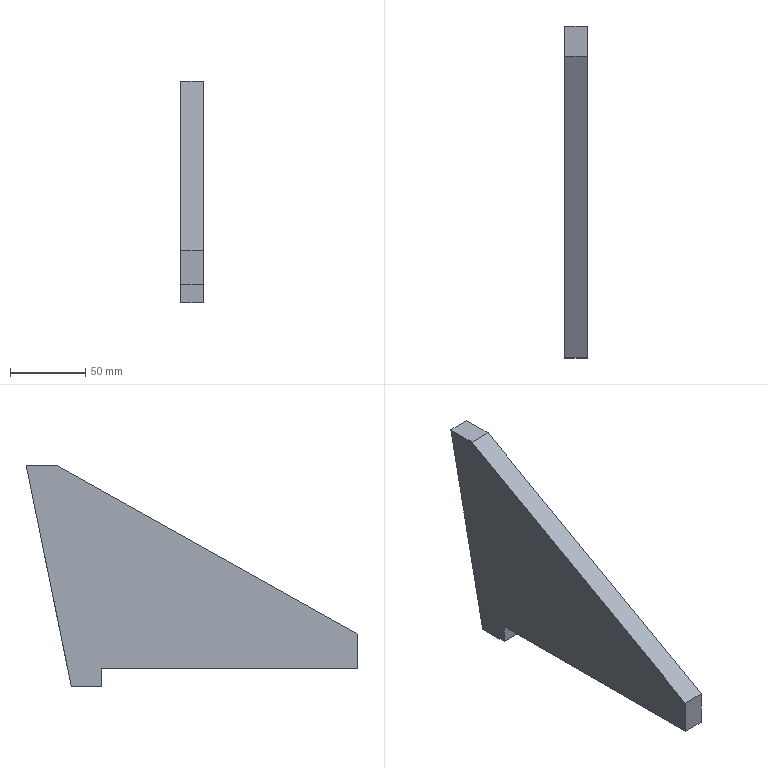Component | SolidWorks | JL001-04-01-003-1 | 1 solid | 41 faces | box 15 x 220 x 147 mm | volume 250990 mm3 | cylinder 16 | cone 16 | plane 9 | commonest cylinder face diameters 5 x16
build123d program:
from build123d import *

# Parameters (mm, degrees)
BOSS_EXTRUDE1_DEPTH   = 7.5
SKETCH2_W             = 12
SKETCH2_H             = 170
CUT_EXTRUDE1_DEPTH    = 266.017
M6_TAPPED_HOLE1_D     = 5
M6_TAPPED_HOLE1_DEPTH = 15
M6_TAPPED_HOLE1_TIP   = 1.502
M6_TAPPED_HOLE2_D     = 5
M6_TAPPED_HOLE2_DEPTH = 15
M6_TAPPED_HOLE2_TIP   = 1.502


with BuildPart() as part:
    # Sketch1 → Boss-Extrude1 (new, symmetric)
    with BuildSketch(Plane(origin=(0, 0, 0), x_dir=(0, 0, -1), z_dir=(1, 0, 0))):
        Polygon((0, 0), (0, -220), (-35, -220), (-147, -20), (-147, 0), align=None)
    extrude(amount=BOSS_EXTRUDE1_DEPTH, both=True)

    # Sketch2 → Cut-Extrude1 (cut, through all)
    with BuildSketch(Plane(origin=(7.5, 0, 0), x_dir=(0, 0, -1), z_dir=(1, 0, 0))):
        Polygon((-147, 0), (0, -30), (0, 0), align=None)
        with Locations((-6, -135)):
            Rectangle(SKETCH2_W, SKETCH2_H)
    extrude(amount=-CUT_EXTRUDE1_DEPTH, mode=Mode.SUBTRACT)

    # M6 Tapped Hole1
    with Locations(Plane(origin=(0, 0, 12), x_dir=(-1, 0, 0), z_dir=(0, 0, -1))):
        with Locations((0, -60), (0, -135), (0, -210), (0, -100), (0, -170)):
            Hole(M6_TAPPED_HOLE1_D / 2, depth=M6_TAPPED_HOLE1_DEPTH)
            with Locations((0, 0, -(M6_TAPPED_HOLE1_DEPTH + M6_TAPPED_HOLE1_TIP / 2))):  # 118° drill point
                Cone(0, M6_TAPPED_HOLE1_D / 2, M6_TAPPED_HOLE1_TIP, mode=Mode.SUBTRACT)

    # M6 Tapped Hole2
    with Locations(Plane(origin=(0, -28.8, 5.878), x_dir=(1, 0, 0), z_dir=(0, 0.9798, -0.2))):
        with Locations((0, -134.016), (0, -69.016), (0, -4.016)):
            Hole(M6_TAPPED_HOLE2_D / 2, depth=M6_TAPPED_HOLE2_DEPTH)
            with Locations((0, 0, -(M6_TAPPED_HOLE2_DEPTH + M6_TAPPED_HOLE2_TIP / 2))):  # 118° drill point
                Cone(0, M6_TAPPED_HOLE2_D / 2, M6_TAPPED_HOLE2_TIP, mode=Mode.SUBTRACT)


solid = part.part

# Placed as in the assembly
solid = solid.moved(Location((142.5, 135, 0), (0, 0, 0)))
STEP:
#1=COLOUR_RGB('',0.7922,0.8196,0.9333);
#2=FILL_AREA_STYLE_COLOUR('',#1);
#3=FILL_AREA_STYLE('',(#2));
#4=SURFACE_STYLE_FILL_AREA(#3);
#5=SURFACE_SIDE_STYLE('',(#4));
#6=SURFACE_STYLE_USAGE(.BOTH.,#5);
#7=PRESENTATION_STYLE_ASSIGNMENT((#6));
#8=CARTESIAN_POINT('',(5.61,4.638,5.423));
#9=VERTEX_POINT('',#8);
#10=CARTESIAN_POINT('',(5.61,4.677,5.616));
#11=VERTEX_POINT('',#10);
#12=CARTESIAN_POINT('',(5.61,4.657,5.519));
#13=DIRECTION('',(0.,0.9798,-0.2));
#14=DIRECTION('',(0.,0.2,0.9798));
#15=AXIS2_PLACEMENT_3D('',#12,#13,#14);
#16=CIRCLE('',#15,0.09843);
#17=EDGE_CURVE('',#9,#11,#16,.T.);
#18=ORIENTED_EDGE('',*,*,#17,.F.);
#19=CARTESIAN_POINT('',(5.61,5.216,5.305));
#20=VERTEX_POINT('',#19);
#21=CARTESIAN_POINT('',(5.61,5.216,5.305));
#22=DIRECTION('',(0.,0.9798,-0.2));
#23=VECTOR('',#22,39.37);
#24=LINE('',#21,#23);
#25=EDGE_CURVE('',#9,#20,#24,.T.);
#26=ORIENTED_EDGE('',*,*,#25,.T.);
#27=CARTESIAN_POINT('',(5.61,5.256,5.498));
#28=VERTEX_POINT('',#27);
#29=CARTESIAN_POINT('',(5.61,5.236,5.401));
#30=DIRECTION('',(0.,0.9798,-0.2));
#31=DIRECTION('',(0.,0.2,0.9798));
#32=AXIS2_PLACEMENT_3D('',#29,#30,#31);
#33=CIRCLE('',#32,0.09843);
#34=EDGE_CURVE('',#20,#28,#33,.T.);
#35=ORIENTED_EDGE('',*,*,#34,.T.);
#36=CARTESIAN_POINT('',(5.61,5.256,5.498));
#37=DIRECTION('',(0.,0.9798,-0.2));
#38=VECTOR('',#37,39.37);
#39=LINE('',#36,#38);
#40=EDGE_CURVE('',#11,#28,#39,.T.);
#41=ORIENTED_EDGE('',*,*,#40,.F.);
#42=EDGE_LOOP('',(#18,#26,#35,#41));
#43=FACE_OUTER_BOUND('',#42,.T.);
#44=CARTESIAN_POINT('',(5.61,5.236,5.401));
#45=DIRECTION('',(0.,0.9798,-0.2));
#46=DIRECTION('',(0.,0.2,0.9798));
#47=AXIS2_PLACEMENT_3D('',#44,#45,#46);
#48=CYLINDRICAL_SURFACE('',#47,0.09843);
#49=ADVANCED_FACE('',(#43),#48,.F.);
#50=CARTESIAN_POINT('',(5.61,4.6,5.531));
#51=VERTEX_POINT('',#50);
#52=CARTESIAN_POINT('',(5.61,4.677,5.616));
#53=DIRECTION('',(0.,0.676,0.7369));
#54=VECTOR('',#53,39.37);
#55=LINE('',#52,#54);
#56=EDGE_CURVE('',#51,#11,#55,.T.);
#57=ORIENTED_EDGE('',*,*,#56,.F.);
#58=CARTESIAN_POINT('',(5.61,4.638,5.423));
#59=DIRECTION('',(0.,0.3332,-0.9428));
#60=VECTOR('',#59,39.37);
#61=LINE('',#58,#60);
#62=EDGE_CURVE('',#51,#9,#61,.T.);
#63=ORIENTED_EDGE('',*,*,#62,.T.);
#64=ORIENTED_EDGE('',*,*,#17,.T.);
#65=EDGE_LOOP('',(#57,#63,#64));
#66=FACE_OUTER_BOUND('',#65,.T.);
#67=CARTESIAN_POINT('',(5.61,4.657,5.519));
#68=DIRECTION('',(0.,0.9798,-0.2));
#69=DIRECTION('',(0.,0.2,0.9798));
#70=AXIS2_PLACEMENT_3D('',#67,#68,#69);
#71=CONICAL_SURFACE('',#70,0.09843,1.03);
#72=ADVANCED_FACE('',(#66),#71,.F.);
#73=CARTESIAN_POINT('',(5.61,4.126,2.915));
#74=VERTEX_POINT('',#73);
#75=CARTESIAN_POINT('',(5.61,4.165,3.108));
#76=VERTEX_POINT('',#75);
#77=CARTESIAN_POINT('',(5.61,4.146,3.012));
#78=DIRECTION('',(0.,0.9798,-0.2));
#79=DIRECTION('',(0.,0.2,0.9798));
#80=AXIS2_PLACEMENT_3D('',#77,#78,#79);
#81=CIRCLE('',#80,0.09843);
#82=EDGE_CURVE('',#74,#76,#81,.T.);
#83=ORIENTED_EDGE('',*,*,#82,.F.);
#84=CARTESIAN_POINT('',(5.61,4.705,2.797));
#85=VERTEX_POINT('',#84);
#86=CARTESIAN_POINT('',(5.61,4.705,2.797));
#87=DIRECTION('',(0.,0.9798,-0.2));
#88=VECTOR('',#87,39.37);
#89=LINE('',#86,#88);
#90=EDGE_CURVE('',#74,#85,#89,.T.);
#91=ORIENTED_EDGE('',*,*,#90,.T.);
#92=CARTESIAN_POINT('',(5.61,4.744,2.99));
#93=VERTEX_POINT('',#92);
#94=CARTESIAN_POINT('',(5.61,4.724,2.894));
#95=DIRECTION('',(0.,0.9798,-0.2));
#96=DIRECTION('',(0.,0.2,0.9798));
#97=AXIS2_PLACEMENT_3D('',#94,#95,#96);
#98=CIRCLE('',#97,0.09843);
#99=EDGE_CURVE('',#85,#93,#98,.T.);
#100=ORIENTED_EDGE('',*,*,#99,.T.);
#101=CARTESIAN_POINT('',(5.61,4.744,2.99));
#102=DIRECTION('',(0.,0.9798,-0.2));
#103=VECTOR('',#102,39.37);
#104=LINE('',#101,#103);
#105=EDGE_CURVE('',#76,#93,#104,.T.);
#106=ORIENTED_EDGE('',*,*,#105,.F.);
#107=EDGE_LOOP('',(#83,#91,#100,#106));
#108=FACE_OUTER_BOUND('',#107,.T.);
#109=CARTESIAN_POINT('',(5.61,4.724,2.894));
#110=DIRECTION('',(0.,0.9798,-0.2));
#111=DIRECTION('',(0.,0.2,0.9798));
#112=AXIS2_PLACEMENT_3D('',#109,#110,#111);
#113=CYLINDRICAL_SURFACE('',#112,0.09843);
#114=ADVANCED_FACE('',(#108),#113,.F.);
#115=CARTESIAN_POINT('',(5.61,4.088,3.024));
#116=VERTEX_POINT('',#115);
#117=CARTESIAN_POINT('',(5.61,4.165,3.108));
#118=DIRECTION('',(0.,0.676,0.7369));
#119=VECTOR('',#118,39.37);
#120=LINE('',#117,#119);
#121=EDGE_CURVE('',#116,#76,#120,.T.);
#122=ORIENTED_EDGE('',*,*,#121,.F.);
#123=CARTESIAN_POINT('',(5.61,4.126,2.915));
#124=DIRECTION('',(0.,0.3332,-0.9428));
#125=VECTOR('',#124,39.37);
#126=LINE('',#123,#125);
#127=EDGE_CURVE('',#116,#74,#126,.T.);
#128=ORIENTED_EDGE('',*,*,#127,.T.);
#129=ORIENTED_EDGE('',*,*,#82,.T.);
#130=EDGE_LOOP('',(#122,#128,#129));
#131=FACE_OUTER_BOUND('',#130,.T.);
#132=CARTESIAN_POINT('',(5.61,4.146,3.012));
#133=DIRECTION('',(0.,0.9798,-0.2));
#134=DIRECTION('',(0.,0.2,0.9798));
#135=AXIS2_PLACEMENT_3D('',#132,#133,#134);
#136=CONICAL_SURFACE('',#135,0.09843,1.03);
#137=ADVANCED_FACE('',(#131),#136,.F.);
#138=CARTESIAN_POINT('',(5.61,3.614,0.408));
#139=VERTEX_POINT('',#138);
#140=CARTESIAN_POINT('',(5.61,3.654,0.6009));
#141=VERTEX_POINT('',#140);
#142=CARTESIAN_POINT('',(5.61,3.634,0.5044));
#143=DIRECTION('',(0.,0.9798,-0.2));
#144=DIRECTION('',(0.,0.2,0.9798));
#145=AXIS2_PLACEMENT_3D('',#142,#143,#144);
#146=CIRCLE('',#145,0.09843);
#147=EDGE_CURVE('',#139,#141,#146,.T.);
#148=ORIENTED_EDGE('',*,*,#147,.F.);
#149=CARTESIAN_POINT('',(5.61,4.193,0.2899));
#150=VERTEX_POINT('',#149);
#151=CARTESIAN_POINT('',(5.61,4.193,0.2899));
#152=DIRECTION('',(0.,0.9798,-0.2));
#153=VECTOR('',#152,39.37);
#154=LINE('',#151,#153);
#155=EDGE_CURVE('',#139,#150,#154,.T.);
#156=ORIENTED_EDGE('',*,*,#155,.T.);
#157=CARTESIAN_POINT('',(5.61,4.232,0.4828));
#158=VERTEX_POINT('',#157);
#159=CARTESIAN_POINT('',(5.61,4.213,0.3863));
#160=DIRECTION('',(0.,0.9798,-0.2));
#161=DIRECTION('',(0.,0.2,0.9798));
#162=AXIS2_PLACEMENT_3D('',#159,#160,#161);
#163=CIRCLE('',#162,0.09843);
#164=EDGE_CURVE('',#150,#158,#163,.T.);
#165=ORIENTED_EDGE('',*,*,#164,.T.);
#166=CARTESIAN_POINT('',(5.61,4.232,0.4828));
#167=DIRECTION('',(0.,0.9798,-0.2));
#168=VECTOR('',#167,39.37);
#169=LINE('',#166,#168);
#170=EDGE_CURVE('',#141,#158,#169,.T.);
#171=ORIENTED_EDGE('',*,*,#170,.F.);
#172=EDGE_LOOP('',(#148,#156,#165,#171));
#173=FACE_OUTER_BOUND('',#172,.T.);
#174=CARTESIAN_POINT('',(5.61,4.213,0.3863));
#175=DIRECTION('',(0.,0.9798,-0.2));
#176=DIRECTION('',(0.,0.2,0.9798));
#177=AXIS2_PLACEMENT_3D('',#174,#175,#176);
#178=CYLINDRICAL_SURFACE('',#177,0.09843);
#179=ADVANCED_FACE('',(#173),#178,.F.);
#180=CARTESIAN_POINT('',(5.61,3.576,0.5162));
#181=VERTEX_POINT('',#180);
#182=CARTESIAN_POINT('',(5.61,3.654,0.6009));
#183=DIRECTION('',(0.,0.676,0.7369));
#184=VECTOR('',#183,39.37);
#185=LINE('',#182,#184);
#186=EDGE_CURVE('',#181,#141,#185,.T.);
#187=ORIENTED_EDGE('',*,*,#186,.F.);
#188=CARTESIAN_POINT('',(5.61,3.614,0.408));
#189=DIRECTION('',(0.,0.3332,-0.9428));
#190=VECTOR('',#189,39.37);
#191=LINE('',#188,#190);
#192=EDGE_CURVE('',#181,#139,#191,.T.);
#193=ORIENTED_EDGE('',*,*,#192,.T.);
#194=ORIENTED_EDGE('',*,*,#147,.T.);
#195=EDGE_LOOP('',(#187,#193,#194));
#196=FACE_OUTER_BOUND('',#195,.T.);
#197=CARTESIAN_POINT('',(5.61,3.634,0.5044));
#198=DIRECTION('',(0.,0.9798,-0.2));
#199=DIRECTION('',(0.,0.2,0.9798));
#200=AXIS2_PLACEMENT_3D('',#197,#198,#199);
#201=CONICAL_SURFACE('',#200,0.09843,1.03);
#202=ADVANCED_FACE('',(#196),#201,.F.);
#203=CARTESIAN_POINT('',(5.61,2.854,1.063));
#204=VERTEX_POINT('',#203);
#205=CARTESIAN_POINT('',(5.61,3.051,1.063));
#206=VERTEX_POINT('',#205);
#207=CARTESIAN_POINT('',(5.61,2.953,1.063));
#208=DIRECTION('',(0.,0.,-1.));
#209=DIRECTION('',(0.,1.,0.));
#210=AXIS2_PLACEMENT_3D('',#207,#208,#209);
#211=CIRCLE('',#210,0.09843);
#212=EDGE_CURVE('',#204,#206,#211,.T.);
#213=ORIENTED_EDGE('',*,*,#212,.F.);
#214=CARTESIAN_POINT('',(5.61,2.854,0.4724));
#215=VERTEX_POINT('',#214);
#216=CARTESIAN_POINT('',(5.61,2.854,0.4724));
#217=DIRECTION('',(0.,0.,-1.));
#218=VECTOR('',#217,39.37);
#219=LINE('',#216,#218);
#220=EDGE_CURVE('',#204,#215,#219,.T.);
#221=ORIENTED_EDGE('',*,*,#220,.T.);
#222=CARTESIAN_POINT('',(5.61,3.051,0.4724));
#223=VERTEX_POINT('',#222);
#224=CARTESIAN_POINT('',(5.61,2.953,0.4724));
#225=DIRECTION('',(0.,0.,-1.));
#226=DIRECTION('',(0.,1.,0.));
#227=AXIS2_PLACEMENT_3D('',#224,#225,#226);
#228=CIRCLE('',#227,0.09843);
#229=EDGE_CURVE('',#215,#223,#228,.T.);
#230=ORIENTED_EDGE('',*,*,#229,.T.);
#231=CARTESIAN_POINT('',(5.61,3.051,0.4724));
#232=DIRECTION('',(0.,0.,-1.));
#233=VECTOR('',#232,39.37);
#234=LINE('',#231,#233);
#235=EDGE_CURVE('',#206,#223,#234,.T.);
#236=ORIENTED_EDGE('',*,*,#235,.F.);
#237=EDGE_LOOP('',(#213,#221,#230,#236));
#238=FACE_OUTER_BOUND('',#237,.T.);
#239=CARTESIAN_POINT('',(5.61,2.953,0.4724));
#240=DIRECTION('',(0.,0.,-1.));
#241=DIRECTION('',(0.,1.,0.));
#242=AXIS2_PLACEMENT_3D('',#239,#240,#241);
#243=CYLINDRICAL_SURFACE('',#242,0.09843);
#244=ADVANCED_FACE('',(#238),#243,.F.);
#245=CARTESIAN_POINT('',(5.61,2.953,1.122));
#246=VERTEX_POINT('',#245);
#247=CARTESIAN_POINT('',(5.61,3.051,1.063));
#248=DIRECTION('',(0.,0.8572,-0.515));
#249=VECTOR('',#248,39.37);
#250=LINE('',#247,#249);
#251=EDGE_CURVE('',#246,#206,#250,.T.);
#252=ORIENTED_EDGE('',*,*,#251,.F.);
#253=CARTESIAN_POINT('',(5.61,2.854,1.063));
#254=DIRECTION('',(0.,-0.8572,-0.515));
#255=VECTOR('',#254,39.37);
#256=LINE('',#253,#255);
#257=EDGE_CURVE('',#246,#204,#256,.T.);
#258=ORIENTED_EDGE('',*,*,#257,.T.);
#259=ORIENTED_EDGE('',*,*,#212,.T.);
#260=EDGE_LOOP('',(#252,#258,#259));
#261=FACE_OUTER_BOUND('',#260,.T.);
#262=CARTESIAN_POINT('',(5.61,2.953,1.063));
#263=DIRECTION('',(0.,0.,-1.));
#264=DIRECTION('',(0.,1.,0.));
#265=AXIS2_PLACEMENT_3D('',#262,#263,#264);
#266=CONICAL_SURFACE('',#265,0.09843,1.03);
#267=ADVANCED_FACE('',(#261),#266,.F.);
#268=CARTESIAN_POINT('',(5.61,-0.09843,1.063));
#269=VERTEX_POINT('',#268);
#270=CARTESIAN_POINT('',(5.61,0.09843,1.063));
#271=VERTEX_POINT('',#270);
#272=CARTESIAN_POINT('',(5.61,0.,1.063));
#273=DIRECTION('',(0.,0.,-1.));
#274=DIRECTION('',(0.,1.,0.));
#275=AXIS2_PLACEMENT_3D('',#272,#273,#274);
#276=CIRCLE('',#275,0.09843);
#277=EDGE_CURVE('',#269,#271,#276,.T.);
#278=ORIENTED_EDGE('',*,*,#277,.F.);
#279=CARTESIAN_POINT('',(5.61,-0.09843,0.4724));
#280=VERTEX_POINT('',#279);
#281=CARTESIAN_POINT('',(5.61,-0.09843,0.4724));
#282=DIRECTION('',(0.,0.,-1.));
#283=VECTOR('',#282,39.37);
#284=LINE('',#281,#283);
#285=EDGE_CURVE('',#269,#280,#284,.T.);
#286=ORIENTED_EDGE('',*,*,#285,.T.);
#287=CARTESIAN_POINT('',(5.61,0.09843,0.4724));
#288=VERTEX_POINT('',#287);
#289=CARTESIAN_POINT('',(5.61,0.,0.4724));
#290=DIRECTION('',(0.,0.,-1.));
#291=DIRECTION('',(0.,1.,0.));
#292=AXIS2_PLACEMENT_3D('',#289,#290,#291);
#293=CIRCLE('',#292,0.09843);
#294=EDGE_CURVE('',#280,#288,#293,.T.);
#295=ORIENTED_EDGE('',*,*,#294,.T.);
#296=CARTESIAN_POINT('',(5.61,0.09843,0.4724));
#297=DIRECTION('',(0.,0.,-1.));
#298=VECTOR('',#297,39.37);
#299=LINE('',#296,#298);
#300=EDGE_CURVE('',#271,#288,#299,.T.);
#301=ORIENTED_EDGE('',*,*,#300,.F.);
#302=EDGE_LOOP('',(#278,#286,#295,#301));
#303=FACE_OUTER_BOUND('',#302,.T.);
#304=CARTESIAN_POINT('',(5.61,0.,0.4724));
#305=DIRECTION('',(0.,0.,-1.));
#306=DIRECTION('',(0.,1.,0.));
#307=AXIS2_PLACEMENT_3D('',#304,#305,#306);
#308=CYLINDRICAL_SURFACE('',#307,0.09843);
#309=ADVANCED_FACE('',(#303),#308,.F.);
#310=CARTESIAN_POINT('',(5.61,0.,1.122));
#311=VERTEX_POINT('',#310);
#312=CARTESIAN_POINT('',(5.61,0.09843,1.063));
#313=DIRECTION('',(0.,0.8572,-0.515));
#314=VECTOR('',#313,39.37);
#315=LINE('',#312,#314);
#316=EDGE_CURVE('',#311,#271,#315,.T.);
#317=ORIENTED_EDGE('',*,*,#316,.F.);
#318=CARTESIAN_POINT('',(5.61,-0.09843,1.063));
#319=DIRECTION('',(0.,-0.8572,-0.515));
#320=VECTOR('',#319,39.37);
#321=LINE('',#318,#320);
#322=EDGE_CURVE('',#311,#269,#321,.T.);
#323=ORIENTED_EDGE('',*,*,#322,.T.);
#324=ORIENTED_EDGE('',*,*,#277,.T.);
#325=EDGE_LOOP('',(#317,#323,#324));
#326=FACE_OUTER_BOUND('',#325,.T.);
#327=CARTESIAN_POINT('',(5.61,0.,1.063));
#328=DIRECTION('',(0.,0.,-1.));
#329=DIRECTION('',(0.,1.,0.));
#330=AXIS2_PLACEMENT_3D('',#327,#328,#329);
#331=CONICAL_SURFACE('',#330,0.09843,1.03);
#332=ADVANCED_FACE('',(#326),#331,.F.);
#333=CARTESIAN_POINT('',(5.61,-3.051,1.063));
#334=VERTEX_POINT('',#333);
#335=CARTESIAN_POINT('',(5.61,-2.854,1.063));
#336=VERTEX_POINT('',#335);
#337=CARTESIAN_POINT('',(5.61,-2.953,1.063));
#338=DIRECTION('',(0.,0.,-1.));
#339=DIRECTION('',(0.,1.,0.));
#340=AXIS2_PLACEMENT_3D('',#337,#338,#339);
#341=CIRCLE('',#340,0.09843);
#342=EDGE_CURVE('',#334,#336,#341,.T.);
#343=ORIENTED_EDGE('',*,*,#342,.F.);
#344=CARTESIAN_POINT('',(5.61,-3.051,0.4724));
#345=VERTEX_POINT('',#344);
#346=CARTESIAN_POINT('',(5.61,-3.051,0.4724));
#347=DIRECTION('',(0.,0.,-1.));
#348=VECTOR('',#347,39.37);
#349=LINE('',#346,#348);
#350=EDGE_CURVE('',#334,#345,#349,.T.);
#351=ORIENTED_EDGE('',*,*,#350,.T.);
#352=CARTESIAN_POINT('',(5.61,-2.854,0.4724));
#353=VERTEX_POINT('',#352);
#354=CARTESIAN_POINT('',(5.61,-2.953,0.4724));
#355=DIRECTION('',(0.,0.,-1.));
#356=DIRECTION('',(0.,1.,0.));
#357=AXIS2_PLACEMENT_3D('',#354,#355,#356);
#358=CIRCLE('',#357,0.09843);
#359=EDGE_CURVE('',#345,#353,#358,.T.);
#360=ORIENTED_EDGE('',*,*,#359,.T.);
#361=CARTESIAN_POINT('',(5.61,-2.854,0.4724));
#362=DIRECTION('',(0.,0.,-1.));
#363=VECTOR('',#362,39.37);
#364=LINE('',#361,#363);
#365=EDGE_CURVE('',#336,#353,#364,.T.);
#366=ORIENTED_EDGE('',*,*,#365,.F.);
#367=EDGE_LOOP('',(#343,#351,#360,#366));
#368=FACE_OUTER_BOUND('',#367,.T.);
#369=CARTESIAN_POINT('',(5.61,-2.953,0.4724));
#370=DIRECTION('',(0.,0.,-1.));
#371=DIRECTION('',(0.,1.,0.));
#372=AXIS2_PLACEMENT_3D('',#369,#370,#371);
#373=CYLINDRICAL_SURFACE('',#372,0.09843);
#374=ADVANCED_FACE('',(#368),#373,.F.);
#375=CARTESIAN_POINT('',(5.61,-2.953,1.122));
#376=VERTEX_POINT('',#375);
#377=CARTESIAN_POINT('',(5.61,-2.854,1.063));
#378=DIRECTION('',(0.,0.8572,-0.515));
#379=VECTOR('',#378,39.37);
#380=LINE('',#377,#379);
#381=EDGE_CURVE('',#376,#336,#380,.T.);
#382=ORIENTED_EDGE('',*,*,#381,.F.);
#383=CARTESIAN_POINT('',(5.61,-3.051,1.063));
#384=DIRECTION('',(0.,-0.8572,-0.515));
#385=VECTOR('',#384,39.37);
#386=LINE('',#383,#385);
#387=EDGE_CURVE('',#376,#334,#386,.T.);
#388=ORIENTED_EDGE('',*,*,#387,.T.);
#389=ORIENTED_EDGE('',*,*,#342,.T.);
#390=EDGE_LOOP('',(#382,#388,#389));
#391=FACE_OUTER_BOUND('',#390,.T.);
#392=CARTESIAN_POINT('',(5.61,-2.953,1.063));
#393=DIRECTION('',(0.,0.,-1.));
#394=DIRECTION('',(0.,1.,0.));
#395=AXIS2_PLACEMENT_3D('',#392,#393,#394);
#396=CONICAL_SURFACE('',#395,0.09843,1.03);
#397=ADVANCED_FACE('',(#391),#396,.F.);
#398=CARTESIAN_POINT('',(5.61,1.28,1.063));
#399=VERTEX_POINT('',#398);
#400=CARTESIAN_POINT('',(5.61,1.476,1.063));
#401=VERTEX_POINT('',#400);
#402=CARTESIAN_POINT('',(5.61,1.378,1.063));
#403=DIRECTION('',(0.,0.,-1.));
#404=DIRECTION('',(0.,1.,0.));
#405=AXIS2_PLACEMENT_3D('',#402,#403,#404);
#406=CIRCLE('',#405,0.09843);
#407=EDGE_CURVE('',#399,#401,#406,.T.);
#408=ORIENTED_EDGE('',*,*,#407,.F.);
#409=CARTESIAN_POINT('',(5.61,1.28,0.4724));
#410=VERTEX_POINT('',#409);
#411=CARTESIAN_POINT('',(5.61,1.28,0.4724));
#412=DIRECTION('',(0.,0.,-1.));
#413=VECTOR('',#412,39.37);
#414=LINE('',#411,#413);
#415=EDGE_CURVE('',#399,#410,#414,.T.);
#416=ORIENTED_EDGE('',*,*,#415,.T.);
#417=CARTESIAN_POINT('',(5.61,1.476,0.4724));
#418=VERTEX_POINT('',#417);
#419=CARTESIAN_POINT('',(5.61,1.378,0.4724));
#420=DIRECTION('',(0.,0.,-1.));
#421=DIRECTION('',(0.,1.,0.));
#422=AXIS2_PLACEMENT_3D('',#419,#420,#421);
#423=CIRCLE('',#422,0.09843);
#424=EDGE_CURVE('',#410,#418,#423,.T.);
#425=ORIENTED_EDGE('',*,*,#424,.T.);
#426=CARTESIAN_POINT('',(5.61,1.476,0.4724));
#427=DIRECTION('',(0.,0.,-1.));
#428=VECTOR('',#427,39.37);
#429=LINE('',#426,#428);
#430=EDGE_CURVE('',#401,#418,#429,.T.);
#431=ORIENTED_EDGE('',*,*,#430,.F.);
#432=EDGE_LOOP('',(#408,#416,#425,#431));
#433=FACE_OUTER_BOUND('',#432,.T.);
#434=CARTESIAN_POINT('',(5.61,1.378,0.4724));
#435=DIRECTION('',(0.,0.,-1.));
#436=DIRECTION('',(0.,1.,0.));
#437=AXIS2_PLACEMENT_3D('',#434,#435,#436);
#438=CYLINDRICAL_SURFACE('',#437,0.09843);
#439=ADVANCED_FACE('',(#433),#438,.F.);
#440=CARTESIAN_POINT('',(5.61,1.378,1.122));
#441=VERTEX_POINT('',#440);
#442=CARTESIAN_POINT('',(5.61,1.476,1.063));
#443=DIRECTION('',(0.,0.8572,-0.515));
#444=VECTOR('',#443,39.37);
#445=LINE('',#442,#444);
#446=EDGE_CURVE('',#441,#401,#445,.T.);
#447=ORIENTED_EDGE('',*,*,#446,.F.);
#448=CARTESIAN_POINT('',(5.61,1.28,1.063));
#449=DIRECTION('',(0.,-0.8572,-0.515));
#450=VECTOR('',#449,39.37);
#451=LINE('',#448,#450);
#452=EDGE_CURVE('',#441,#399,#451,.T.);
#453=ORIENTED_EDGE('',*,*,#452,.T.);
#454=ORIENTED_EDGE('',*,*,#407,.T.);
#455=EDGE_LOOP('',(#447,#453,#454));
#456=FACE_OUTER_BOUND('',#455,.T.);
#457=CARTESIAN_POINT('',(5.61,1.378,1.063));
#458=DIRECTION('',(0.,0.,-1.));
#459=DIRECTION('',(0.,1.,0.));
#460=AXIS2_PLACEMENT_3D('',#457,#458,#459);
#461=CONICAL_SURFACE('',#460,0.09843,1.03);
#462=ADVANCED_FACE('',(#456),#461,.F.);
#463=CARTESIAN_POINT('',(5.61,-1.476,1.063));
#464=VERTEX_POINT('',#463);
#465=CARTESIAN_POINT('',(5.61,-1.28,1.063));
#466=VERTEX_POINT('',#465);
#467=CARTESIAN_POINT('',(5.61,-1.378,1.063));
#468=DIRECTION('',(0.,0.,-1.));
#469=DIRECTION('',(0.,1.,0.));
#470=AXIS2_PLACEMENT_3D('',#467,#468,#469);
#471=CIRCLE('',#470,0.09843);
#472=EDGE_CURVE('',#464,#466,#471,.T.);
#473=ORIENTED_EDGE('',*,*,#472,.F.);
#474=CARTESIAN_POINT('',(5.61,-1.476,0.4724));
#475=VERTEX_POINT('',#474);
#476=CARTESIAN_POINT('',(5.61,-1.476,0.4724));
#477=DIRECTION('',(0.,0.,-1.));
#478=VECTOR('',#477,39.37);
#479=LINE('',#476,#478);
#480=EDGE_CURVE('',#464,#475,#479,.T.);
#481=ORIENTED_EDGE('',*,*,#480,.T.);
#482=CARTESIAN_POINT('',(5.61,-1.28,0.4724));
#483=VERTEX_POINT('',#482);
#484=CARTESIAN_POINT('',(5.61,-1.378,0.4724));
#485=DIRECTION('',(0.,0.,-1.));
#486=DIRECTION('',(0.,1.,0.));
#487=AXIS2_PLACEMENT_3D('',#484,#485,#486);
#488=CIRCLE('',#487,0.09843);
#489=EDGE_CURVE('',#475,#483,#488,.T.);
#490=ORIENTED_EDGE('',*,*,#489,.T.);
#491=CARTESIAN_POINT('',(5.61,-1.28,0.4724));
#492=DIRECTION('',(0.,0.,-1.));
#493=VECTOR('',#492,39.37);
#494=LINE('',#491,#493);
#495=EDGE_CURVE('',#466,#483,#494,.T.);
#496=ORIENTED_EDGE('',*,*,#495,.F.);
#497=EDGE_LOOP('',(#473,#481,#490,#496));
#498=FACE_OUTER_BOUND('',#497,.T.);
#499=CARTESIAN_POINT('',(5.61,-1.378,0.4724));
#500=DIRECTION('',(0.,0.,-1.));
#501=DIRECTION('',(0.,1.,0.));
#502=AXIS2_PLACEMENT_3D('',#499,#500,#501);
#503=CYLINDRICAL_SURFACE('',#502,0.09843);
#504=ADVANCED_FACE('',(#498),#503,.F.);
#505=CARTESIAN_POINT('',(5.61,-1.378,1.122));
#506=VERTEX_POINT('',#505);
#507=CARTESIAN_POINT('',(5.61,-1.28,1.063));
#508=DIRECTION('',(0.,0.8572,-0.515));
#509=VECTOR('',#508,39.37);
#510=LINE('',#507,#509);
#511=EDGE_CURVE('',#506,#466,#510,.T.);
#512=ORIENTED_EDGE('',*,*,#511,.F.);
#513=CARTESIAN_POINT('',(5.61,-1.476,1.063));
#514=DIRECTION('',(0.,-0.8572,-0.515));
#515=VECTOR('',#514,39.37);
#516=LINE('',#513,#515);
#517=EDGE_CURVE('',#506,#464,#516,.T.);
#518=ORIENTED_EDGE('',*,*,#517,.T.);
#519=ORIENTED_EDGE('',*,*,#472,.T.);
#520=EDGE_LOOP('',(#512,#518,#519));
#521=FACE_OUTER_BOUND('',#520,.T.);
#522=CARTESIAN_POINT('',(5.61,-1.378,1.063));
#523=DIRECTION('',(0.,0.,-1.));
#524=DIRECTION('',(0.,1.,0.));
#525=AXIS2_PLACEMENT_3D('',#522,#523,#524);
#526=CONICAL_SURFACE('',#525,0.09843,1.03);
#527=ADVANCED_FACE('',(#521),#526,.F.);
#528=CARTESIAN_POINT('',(5.315,5.315,5.787));
#529=VERTEX_POINT('',#528);
#530=CARTESIAN_POINT('',(5.315,4.528,5.787));
#531=VERTEX_POINT('',#530);
#532=CARTESIAN_POINT('',(5.315,4.528,5.787));
#533=DIRECTION('',(0.,-1.,0.));
#534=VECTOR('',#533,39.37);
#535=LINE('',#532,#534);
#536=EDGE_CURVE('',#529,#531,#535,.T.);
#537=ORIENTED_EDGE('',*,*,#536,.T.);
#538=CARTESIAN_POINT('',(5.906,4.528,5.787));
#539=VERTEX_POINT('',#538);
#540=CARTESIAN_POINT('',(5.906,4.528,5.787));
#541=DIRECTION('',(-1.,0.,0.));
#542=VECTOR('',#541,39.37);
#543=LINE('',#540,#542);
#544=EDGE_CURVE('',#539,#531,#543,.T.);
#545=ORIENTED_EDGE('',*,*,#544,.F.);
#546=CARTESIAN_POINT('',(5.906,5.315,5.787));
#547=VERTEX_POINT('',#546);
#548=CARTESIAN_POINT('',(5.906,4.528,5.787));
#549=DIRECTION('',(0.,-1.,0.));
#550=VECTOR('',#549,39.37);
#551=LINE('',#548,#550);
#552=EDGE_CURVE('',#547,#539,#551,.T.);
#553=ORIENTED_EDGE('',*,*,#552,.F.);
#554=CARTESIAN_POINT('',(5.906,5.315,5.787));
#555=DIRECTION('',(-1.,0.,0.));
#556=VECTOR('',#555,39.37);
#557=LINE('',#554,#556);
#558=EDGE_CURVE('',#547,#529,#557,.T.);
#559=ORIENTED_EDGE('',*,*,#558,.T.);
#560=EDGE_LOOP('',(#537,#545,#553,#559));
#561=FACE_OUTER_BOUND('',#560,.T.);
#562=CARTESIAN_POINT('',(5.906,4.528,5.787));
#563=DIRECTION('',(0.,0.,-1.));
#564=DIRECTION('',(-1.,0.,0.));
#565=AXIS2_PLACEMENT_3D('',#562,#563,#564);
#566=PLANE('',#565);
#567=ADVANCED_FACE('',(#561),#566,.F.);
#568=CARTESIAN_POINT('',(5.315,-3.346,1.378));
#569=VERTEX_POINT('',#568);
#570=CARTESIAN_POINT('',(5.315,-3.346,1.378));
#571=DIRECTION('',(0.,-0.8725,-0.4886));
#572=VECTOR('',#571,39.37);
#573=LINE('',#570,#572);
#574=EDGE_CURVE('',#531,#569,#573,.T.);
#575=ORIENTED_EDGE('',*,*,#574,.T.);
#576=CARTESIAN_POINT('',(5.906,-3.346,1.378));
#577=VERTEX_POINT('',#576);
#578=CARTESIAN_POINT('',(5.906,-3.346,1.378));
#579=DIRECTION('',(-1.,0.,0.));
#580=VECTOR('',#579,39.37);
#581=LINE('',#578,#580);
#582=EDGE_CURVE('',#577,#569,#581,.T.);
#583=ORIENTED_EDGE('',*,*,#582,.F.);
#584=CARTESIAN_POINT('',(5.906,-3.346,1.378));
#585=DIRECTION('',(0.,-0.8725,-0.4886));
#586=VECTOR('',#585,39.37);
#587=LINE('',#584,#586);
#588=EDGE_CURVE('',#539,#577,#587,.T.);
#589=ORIENTED_EDGE('',*,*,#588,.F.);
#590=ORIENTED_EDGE('',*,*,#544,.T.);
#591=EDGE_LOOP('',(#575,#583,#589,#590));
#592=FACE_OUTER_BOUND('',#591,.T.);
#593=CARTESIAN_POINT('',(5.906,-3.346,1.378));
#594=DIRECTION('',(0.,0.4886,-0.8725));
#595=DIRECTION('',(0.,0.8725,0.4886));
#596=AXIS2_PLACEMENT_3D('',#593,#594,#595);
#597=PLANE('',#596);
#598=ADVANCED_FACE('',(#592),#597,.F.);
#599=CARTESIAN_POINT('',(5.315,-3.346,0.4724));
#600=VERTEX_POINT('',#599);
#601=CARTESIAN_POINT('',(5.315,-3.346,-0.));
#602=DIRECTION('',(0.,0.,-1.));
#603=VECTOR('',#602,39.37);
#604=LINE('',#601,#603);
#605=EDGE_CURVE('',#569,#600,#604,.T.);
#606=ORIENTED_EDGE('',*,*,#605,.T.);
#607=CARTESIAN_POINT('',(5.906,-3.346,0.4724));
#608=VERTEX_POINT('',#607);
#609=CARTESIAN_POINT('',(5.315,-3.346,0.4724));
#610=DIRECTION('',(1.,0.,0.));
#611=VECTOR('',#610,39.37);
#612=LINE('',#609,#611);
#613=EDGE_CURVE('',#600,#608,#612,.T.);
#614=ORIENTED_EDGE('',*,*,#613,.T.);
#615=CARTESIAN_POINT('',(5.906,-3.346,-0.));
#616=DIRECTION('',(0.,0.,-1.));
#617=VECTOR('',#616,39.37);
#618=LINE('',#615,#617);
#619=EDGE_CURVE('',#577,#608,#618,.T.);
#620=ORIENTED_EDGE('',*,*,#619,.F.);
#621=ORIENTED_EDGE('',*,*,#582,.T.);
#622=EDGE_LOOP('',(#606,#614,#620,#621));
#623=FACE_OUTER_BOUND('',#622,.T.);
#624=CARTESIAN_POINT('',(5.906,-3.346,-0.));
#625=DIRECTION('',(0.,1.,0.));
#626=DIRECTION('',(0.,0.,1.));
#627=AXIS2_PLACEMENT_3D('',#624,#625,#626);
#628=PLANE('',#627);
#629=ADVANCED_FACE('',(#623),#628,.F.);
#630=CARTESIAN_POINT('',(5.906,3.346,-0.));
#631=VERTEX_POINT('',#630);
#632=CARTESIAN_POINT('',(5.906,4.134,-0.));
#633=VERTEX_POINT('',#632);
#634=CARTESIAN_POINT('',(5.906,5.315,0.));
#635=DIRECTION('',(0.,1.,0.));
#636=VECTOR('',#635,39.37);
#637=LINE('',#634,#636);
#638=EDGE_CURVE('',#631,#633,#637,.T.);
#639=ORIENTED_EDGE('',*,*,#638,.F.);
#640=CARTESIAN_POINT('',(5.315,3.346,-0.));
#641=VERTEX_POINT('',#640);
#642=CARTESIAN_POINT('',(5.315,3.346,-0.));
#643=DIRECTION('',(1.,0.,0.));
#644=VECTOR('',#643,39.37);
#645=LINE('',#642,#644);
#646=EDGE_CURVE('',#641,#631,#645,.T.);
#647=ORIENTED_EDGE('',*,*,#646,.F.);
#648=CARTESIAN_POINT('',(5.315,4.134,0.));
#649=VERTEX_POINT('',#648);
#650=CARTESIAN_POINT('',(5.315,5.315,0.));
#651=DIRECTION('',(0.,1.,0.));
#652=VECTOR('',#651,39.37);
#653=LINE('',#650,#652);
#654=EDGE_CURVE('',#641,#649,#653,.T.);
#655=ORIENTED_EDGE('',*,*,#654,.T.);
#656=CARTESIAN_POINT('',(5.315,4.134,-0.));
#657=DIRECTION('',(1.,0.,0.));
#658=VECTOR('',#657,39.37);
#659=LINE('',#656,#658);
#660=EDGE_CURVE('',#649,#633,#659,.T.);
#661=ORIENTED_EDGE('',*,*,#660,.T.);
#662=EDGE_LOOP('',(#639,#647,#655,#661));
#663=FACE_OUTER_BOUND('',#662,.T.);
#664=CARTESIAN_POINT('',(5.906,5.315,0.));
#665=DIRECTION('',(0.,-0.,1.));
#666=DIRECTION('',(0.,-1.,-0.));
#667=AXIS2_PLACEMENT_3D('',#664,#665,#666);
#668=PLANE('',#667);
#669=ADVANCED_FACE('',(#663),#668,.F.);
#670=ORIENTED_EDGE('',*,*,#619,.T.);
#671=CARTESIAN_POINT('',(5.906,3.346,0.4724));
#672=VERTEX_POINT('',#671);
#673=CARTESIAN_POINT('',(5.906,3.346,0.4724));
#674=DIRECTION('',(0.,-1.,-0.));
#675=VECTOR('',#674,39.37);
#676=LINE('',#673,#675);
#677=EDGE_CURVE('',#672,#608,#676,.T.);
#678=ORIENTED_EDGE('',*,*,#677,.F.);
#679=CARTESIAN_POINT('',(5.906,3.346,-0.));
#680=DIRECTION('',(0.,0.,1.));
#681=VECTOR('',#680,39.37);
#682=LINE('',#679,#681);
#683=EDGE_CURVE('',#631,#672,#682,.T.);
#684=ORIENTED_EDGE('',*,*,#683,.F.);
#685=ORIENTED_EDGE('',*,*,#638,.T.);
#686=CARTESIAN_POINT('',(5.906,5.315,5.787));
#687=DIRECTION('',(0.,-0.2,-0.9798));
#688=VECTOR('',#687,39.37);
#689=LINE('',#686,#688);
#690=EDGE_CURVE('',#547,#633,#689,.T.);
#691=ORIENTED_EDGE('',*,*,#690,.F.);
#692=ORIENTED_EDGE('',*,*,#552,.T.);
#693=ORIENTED_EDGE('',*,*,#588,.T.);
#694=EDGE_LOOP('',(#670,#678,#684,#685,#691,#692,#693));
#695=FACE_OUTER_BOUND('',#694,.T.);
#696=CARTESIAN_POINT('',(5.906,5.315,0.));
#697=DIRECTION('',(-1.,0.,0.));
#698=DIRECTION('',(0.,0.,1.));
#699=AXIS2_PLACEMENT_3D('',#696,#697,#698);
#700=PLANE('',#699);
#701=ADVANCED_FACE('',(#695),#700,.F.);
#702=CARTESIAN_POINT('',(5.315,3.346,0.4724));
#703=VERTEX_POINT('',#702);
#704=CARTESIAN_POINT('',(5.315,3.346,0.4724));
#705=DIRECTION('',(0.,-1.,-0.));
#706=VECTOR('',#705,39.37);
#707=LINE('',#704,#706);
#708=EDGE_CURVE('',#703,#600,#707,.T.);
#709=ORIENTED_EDGE('',*,*,#708,.T.);
#710=ORIENTED_EDGE('',*,*,#605,.F.);
#711=ORIENTED_EDGE('',*,*,#574,.F.);
#712=ORIENTED_EDGE('',*,*,#536,.F.);
#713=CARTESIAN_POINT('',(5.315,5.315,5.787));
#714=DIRECTION('',(0.,-0.2,-0.9798));
#715=VECTOR('',#714,39.37);
#716=LINE('',#713,#715);
#717=EDGE_CURVE('',#529,#649,#716,.T.);
#718=ORIENTED_EDGE('',*,*,#717,.T.);
#719=ORIENTED_EDGE('',*,*,#654,.F.);
#720=CARTESIAN_POINT('',(5.315,3.346,-0.));
#721=DIRECTION('',(0.,0.,1.));
#722=VECTOR('',#721,39.37);
#723=LINE('',#720,#722);
#724=EDGE_CURVE('',#641,#703,#723,.T.);
#725=ORIENTED_EDGE('',*,*,#724,.T.);
#726=EDGE_LOOP('',(#709,#710,#711,#712,#718,#719,#725));
#727=FACE_OUTER_BOUND('',#726,.T.);
#728=CARTESIAN_POINT('',(5.315,5.315,0.));
#729=DIRECTION('',(-1.,0.,0.));
#730=DIRECTION('',(0.,0.,1.));
#731=AXIS2_PLACEMENT_3D('',#728,#729,#730);
#732=PLANE('',#731);
#733=ADVANCED_FACE('',(#727),#732,.T.);
#734=CARTESIAN_POINT('',(5.61,5.236,5.401));
#735=DIRECTION('',(0.,0.9798,-0.2));
#736=DIRECTION('',(0.,0.2,0.9798));
#737=AXIS2_PLACEMENT_3D('',#734,#735,#736);
#738=CIRCLE('',#737,0.09843);
#739=EDGE_CURVE('',#28,#20,#738,.T.);
#740=ORIENTED_EDGE('',*,*,#739,.F.);
#741=ORIENTED_EDGE('',*,*,#34,.F.);
#742=EDGE_LOOP('',(#740,#741));
#743=FACE_BOUND('',#742,.T.);
#744=CARTESIAN_POINT('',(5.61,4.724,2.894));
#745=DIRECTION('',(0.,0.9798,-0.2));
#746=DIRECTION('',(0.,0.2,0.9798));
#747=AXIS2_PLACEMENT_3D('',#744,#745,#746);
#748=CIRCLE('',#747,0.09843);
#749=EDGE_CURVE('',#93,#85,#748,.T.);
#750=ORIENTED_EDGE('',*,*,#749,.F.);
#751=ORIENTED_EDGE('',*,*,#99,.F.);
#752=EDGE_LOOP('',(#750,#751));
#753=FACE_BOUND('',#752,.T.);
#754=CARTESIAN_POINT('',(5.61,4.213,0.3863));
#755=DIRECTION('',(0.,0.9798,-0.2));
#756=DIRECTION('',(0.,0.2,0.9798));
#757=AXIS2_PLACEMENT_3D('',#754,#755,#756);
#758=CIRCLE('',#757,0.09843);
#759=EDGE_CURVE('',#158,#150,#758,.T.);
#760=ORIENTED_EDGE('',*,*,#759,.F.);
#761=ORIENTED_EDGE('',*,*,#164,.F.);
#762=EDGE_LOOP('',(#760,#761));
#763=FACE_BOUND('',#762,.T.);
#764=ORIENTED_EDGE('',*,*,#690,.T.);
#765=ORIENTED_EDGE('',*,*,#660,.F.);
#766=ORIENTED_EDGE('',*,*,#717,.F.);
#767=ORIENTED_EDGE('',*,*,#558,.F.);
#768=EDGE_LOOP('',(#764,#765,#766,#767));
#769=FACE_OUTER_BOUND('',#768,.T.);
#770=CARTESIAN_POINT('',(5.315,5.315,5.787));
#771=DIRECTION('',(0.,-0.9798,0.2));
#772=DIRECTION('',(0.,-0.2,-0.9798));
#773=AXIS2_PLACEMENT_3D('',#770,#771,#772);
#774=PLANE('',#773);
#775=ADVANCED_FACE('',(#743,#753,#763,#769),#774,.F.);
#776=CARTESIAN_POINT('',(5.61,2.953,0.4724));
#777=DIRECTION('',(0.,0.,-1.));
#778=DIRECTION('',(0.,1.,0.));
#779=AXIS2_PLACEMENT_3D('',#776,#777,#778);
#780=CIRCLE('',#779,0.09843);
#781=EDGE_CURVE('',#223,#215,#780,.T.);
#782=ORIENTED_EDGE('',*,*,#781,.F.);
#783=ORIENTED_EDGE('',*,*,#229,.F.);
#784=EDGE_LOOP('',(#782,#783));
#785=FACE_BOUND('',#784,.T.);
#786=CARTESIAN_POINT('',(5.61,0.,0.4724));
#787=DIRECTION('',(0.,0.,-1.));
#788=DIRECTION('',(0.,1.,0.));
#789=AXIS2_PLACEMENT_3D('',#786,#787,#788);
#790=CIRCLE('',#789,0.09843);
#791=EDGE_CURVE('',#288,#280,#790,.T.);
#792=ORIENTED_EDGE('',*,*,#791,.F.);
#793=ORIENTED_EDGE('',*,*,#294,.F.);
#794=EDGE_LOOP('',(#792,#793));
#795=FACE_BOUND('',#794,.T.);
#796=CARTESIAN_POINT('',(5.61,-2.953,0.4724));
#797=DIRECTION('',(0.,0.,-1.));
#798=DIRECTION('',(0.,1.,0.));
#799=AXIS2_PLACEMENT_3D('',#796,#797,#798);
#800=CIRCLE('',#799,0.09843);
#801=EDGE_CURVE('',#353,#345,#800,.T.);
#802=ORIENTED_EDGE('',*,*,#801,.F.);
#803=ORIENTED_EDGE('',*,*,#359,.F.);
#804=EDGE_LOOP('',(#802,#803));
#805=FACE_BOUND('',#804,.T.);
#806=CARTESIAN_POINT('',(5.61,1.378,0.4724));
#807=DIRECTION('',(0.,0.,-1.));
#808=DIRECTION('',(0.,1.,0.));
#809=AXIS2_PLACEMENT_3D('',#806,#807,#808);
#810=CIRCLE('',#809,0.09843);
#811=EDGE_CURVE('',#418,#410,#810,.T.);
#812=ORIENTED_EDGE('',*,*,#811,.F.);
#813=ORIENTED_EDGE('',*,*,#424,.F.);
#814=EDGE_LOOP('',(#812,#813));
#815=FACE_BOUND('',#814,.T.);
#816=CARTESIAN_POINT('',(5.61,-1.378,0.4724));
#817=DIRECTION('',(0.,0.,-1.));
#818=DIRECTION('',(0.,1.,0.));
#819=AXIS2_PLACEMENT_3D('',#816,#817,#818);
#820=CIRCLE('',#819,0.09843);
#821=EDGE_CURVE('',#483,#475,#820,.T.);
#822=ORIENTED_EDGE('',*,*,#821,.F.);
#823=ORIENTED_EDGE('',*,*,#489,.F.);
#824=EDGE_LOOP('',(#822,#823));
#825=FACE_BOUND('',#824,.T.);
#826=ORIENTED_EDGE('',*,*,#677,.T.);
#827=ORIENTED_EDGE('',*,*,#613,.F.);
#828=ORIENTED_EDGE('',*,*,#708,.F.);
#829=CARTESIAN_POINT('',(5.315,3.346,0.4724));
#830=DIRECTION('',(1.,0.,0.));
#831=VECTOR('',#830,39.37);
#832=LINE('',#829,#831);
#833=EDGE_CURVE('',#703,#672,#832,.T.);
#834=ORIENTED_EDGE('',*,*,#833,.T.);
#835=EDGE_LOOP('',(#826,#827,#828,#834));
#836=FACE_OUTER_BOUND('',#835,.T.);
#837=CARTESIAN_POINT('',(5.315,3.346,0.4724));
#838=DIRECTION('',(0.,-0.,1.));
#839=DIRECTION('',(0.,-1.,-0.));
#840=AXIS2_PLACEMENT_3D('',#837,#838,#839);
#841=PLANE('',#840);
#842=ADVANCED_FACE('',(#785,#795,#805,#815,#825,#836),#841,.F.);
#843=ORIENTED_EDGE('',*,*,#683,.T.);
#844=ORIENTED_EDGE('',*,*,#833,.F.);
#845=ORIENTED_EDGE('',*,*,#724,.F.);
#846=ORIENTED_EDGE('',*,*,#646,.T.);
#847=EDGE_LOOP('',(#843,#844,#845,#846));
#848=FACE_OUTER_BOUND('',#847,.T.);
#849=CARTESIAN_POINT('',(5.315,3.346,-0.));
#850=DIRECTION('',(0.,1.,0.));
#851=DIRECTION('',(0.,0.,1.));
#852=AXIS2_PLACEMENT_3D('',#849,#850,#851);
#853=PLANE('',#852);
#854=ADVANCED_FACE('',(#848),#853,.F.);
#855=ORIENTED_EDGE('',*,*,#517,.F.);
#856=ORIENTED_EDGE('',*,*,#511,.T.);
#857=CARTESIAN_POINT('',(5.61,-1.378,1.063));
#858=DIRECTION('',(0.,0.,-1.));
#859=DIRECTION('',(0.,1.,0.));
#860=AXIS2_PLACEMENT_3D('',#857,#858,#859);
#861=CIRCLE('',#860,0.09843);
#862=EDGE_CURVE('',#466,#464,#861,.T.);
#863=ORIENTED_EDGE('',*,*,#862,.T.);
#864=EDGE_LOOP('',(#855,#856,#863));
#865=FACE_OUTER_BOUND('',#864,.T.);
#866=CARTESIAN_POINT('',(5.61,-1.378,1.063));
#867=DIRECTION('',(0.,0.,-1.));
#868=DIRECTION('',(0.,1.,0.));
#869=AXIS2_PLACEMENT_3D('',#866,#867,#868);
#870=CONICAL_SURFACE('',#869,0.09843,1.03);
#871=ADVANCED_FACE('',(#865),#870,.F.);
#872=ORIENTED_EDGE('',*,*,#480,.F.);
#873=ORIENTED_EDGE('',*,*,#862,.F.);
#874=ORIENTED_EDGE('',*,*,#495,.T.);
#875=ORIENTED_EDGE('',*,*,#821,.T.);
#876=EDGE_LOOP('',(#872,#873,#874,#875));
#877=FACE_OUTER_BOUND('',#876,.T.);
#878=CARTESIAN_POINT('',(5.61,-1.378,0.4724));
#879=DIRECTION('',(0.,0.,-1.));
#880=DIRECTION('',(0.,1.,0.));
#881=AXIS2_PLACEMENT_3D('',#878,#879,#880);
#882=CYLINDRICAL_SURFACE('',#881,0.09843);
#883=ADVANCED_FACE('',(#877),#882,.F.);
#884=ORIENTED_EDGE('',*,*,#452,.F.);
#885=ORIENTED_EDGE('',*,*,#446,.T.);
#886=CARTESIAN_POINT('',(5.61,1.378,1.063));
#887=DIRECTION('',(0.,0.,-1.));
#888=DIRECTION('',(0.,1.,0.));
#889=AXIS2_PLACEMENT_3D('',#886,#887,#888);
#890=CIRCLE('',#889,0.09843);
#891=EDGE_CURVE('',#401,#399,#890,.T.);
#892=ORIENTED_EDGE('',*,*,#891,.T.);
#893=EDGE_LOOP('',(#884,#885,#892));
#894=FACE_OUTER_BOUND('',#893,.T.);
#895=CARTESIAN_POINT('',(5.61,1.378,1.063));
#896=DIRECTION('',(0.,0.,-1.));
#897=DIRECTION('',(0.,1.,0.));
#898=AXIS2_PLACEMENT_3D('',#895,#896,#897);
#899=CONICAL_SURFACE('',#898,0.09843,1.03);
#900=ADVANCED_FACE('',(#894),#899,.F.);
#901=ORIENTED_EDGE('',*,*,#415,.F.);
#902=ORIENTED_EDGE('',*,*,#891,.F.);
#903=ORIENTED_EDGE('',*,*,#430,.T.);
#904=ORIENTED_EDGE('',*,*,#811,.T.);
#905=EDGE_LOOP('',(#901,#902,#903,#904));
#906=FACE_OUTER_BOUND('',#905,.T.);
#907=CARTESIAN_POINT('',(5.61,1.378,0.4724));
#908=DIRECTION('',(0.,0.,-1.));
#909=DIRECTION('',(0.,1.,0.));
#910=AXIS2_PLACEMENT_3D('',#907,#908,#909);
#911=CYLINDRICAL_SURFACE('',#910,0.09843);
#912=ADVANCED_FACE('',(#906),#911,.F.);
#913=ORIENTED_EDGE('',*,*,#387,.F.);
#914=ORIENTED_EDGE('',*,*,#381,.T.);
#915=CARTESIAN_POINT('',(5.61,-2.953,1.063));
#916=DIRECTION('',(0.,0.,-1.));
#917=DIRECTION('',(0.,1.,0.));
#918=AXIS2_PLACEMENT_3D('',#915,#916,#917);
#919=CIRCLE('',#918,0.09843);
#920=EDGE_CURVE('',#336,#334,#919,.T.);
#921=ORIENTED_EDGE('',*,*,#920,.T.);
#922=EDGE_LOOP('',(#913,#914,#921));
#923=FACE_OUTER_BOUND('',#922,.T.);
#924=CARTESIAN_POINT('',(5.61,-2.953,1.063));
#925=DIRECTION('',(0.,0.,-1.));
#926=DIRECTION('',(0.,1.,0.));
#927=AXIS2_PLACEMENT_3D('',#924,#925,#926);
#928=CONICAL_SURFACE('',#927,0.09843,1.03);
#929=ADVANCED_FACE('',(#923),#928,.F.);
#930=ORIENTED_EDGE('',*,*,#350,.F.);
#931=ORIENTED_EDGE('',*,*,#920,.F.);
#932=ORIENTED_EDGE('',*,*,#365,.T.);
#933=ORIENTED_EDGE('',*,*,#801,.T.);
#934=EDGE_LOOP('',(#930,#931,#932,#933));
#935=FACE_OUTER_BOUND('',#934,.T.);
#936=CARTESIAN_POINT('',(5.61,-2.953,0.4724));
#937=DIRECTION('',(0.,0.,-1.));
#938=DIRECTION('',(0.,1.,0.));
#939=AXIS2_PLACEMENT_3D('',#936,#937,#938);
#940=CYLINDRICAL_SURFACE('',#939,0.09843);
#941=ADVANCED_FACE('',(#935),#940,.F.);
#942=ORIENTED_EDGE('',*,*,#322,.F.);
#943=ORIENTED_EDGE('',*,*,#316,.T.);
#944=CARTESIAN_POINT('',(5.61,0.,1.063));
#945=DIRECTION('',(0.,0.,-1.));
#946=DIRECTION('',(0.,1.,0.));
#947=AXIS2_PLACEMENT_3D('',#944,#945,#946);
#948=CIRCLE('',#947,0.09843);
#949=EDGE_CURVE('',#271,#269,#948,.T.);
#950=ORIENTED_EDGE('',*,*,#949,.T.);
#951=EDGE_LOOP('',(#942,#943,#950));
#952=FACE_OUTER_BOUND('',#951,.T.);
#953=CARTESIAN_POINT('',(5.61,0.,1.063));
#954=DIRECTION('',(0.,0.,-1.));
#955=DIRECTION('',(0.,1.,0.));
#956=AXIS2_PLACEMENT_3D('',#953,#954,#955);
#957=CONICAL_SURFACE('',#956,0.09843,1.03);
#958=ADVANCED_FACE('',(#952),#957,.F.);
#959=ORIENTED_EDGE('',*,*,#285,.F.);
#960=ORIENTED_EDGE('',*,*,#949,.F.);
#961=ORIENTED_EDGE('',*,*,#300,.T.);
#962=ORIENTED_EDGE('',*,*,#791,.T.);
#963=EDGE_LOOP('',(#959,#960,#961,#962));
#964=FACE_OUTER_BOUND('',#963,.T.);
#965=CARTESIAN_POINT('',(5.61,0.,0.4724));
#966=DIRECTION('',(0.,0.,-1.));
#967=DIRECTION('',(0.,1.,0.));
#968=AXIS2_PLACEMENT_3D('',#965,#966,#967);
#969=CYLINDRICAL_SURFACE('',#968,0.09843);
#970=ADVANCED_FACE('',(#964),#969,.F.);
#971=ORIENTED_EDGE('',*,*,#257,.F.);
#972=ORIENTED_EDGE('',*,*,#251,.T.);
#973=CARTESIAN_POINT('',(5.61,2.953,1.063));
#974=DIRECTION('',(0.,0.,-1.));
#975=DIRECTION('',(0.,1.,0.));
#976=AXIS2_PLACEMENT_3D('',#973,#974,#975);
#977=CIRCLE('',#976,0.09843);
#978=EDGE_CURVE('',#206,#204,#977,.T.);
#979=ORIENTED_EDGE('',*,*,#978,.T.);
#980=EDGE_LOOP('',(#971,#972,#979));
#981=FACE_OUTER_BOUND('',#980,.T.);
#982=CARTESIAN_POINT('',(5.61,2.953,1.063));
#983=DIRECTION('',(0.,0.,-1.));
#984=DIRECTION('',(0.,1.,0.));
#985=AXIS2_PLACEMENT_3D('',#982,#983,#984);
#986=CONICAL_SURFACE('',#985,0.09843,1.03);
#987=ADVANCED_FACE('',(#981),#986,.F.);
#988=ORIENTED_EDGE('',*,*,#220,.F.);
#989=ORIENTED_EDGE('',*,*,#978,.F.);
#990=ORIENTED_EDGE('',*,*,#235,.T.);
#991=ORIENTED_EDGE('',*,*,#781,.T.);
#992=EDGE_LOOP('',(#988,#989,#990,#991));
#993=FACE_OUTER_BOUND('',#992,.T.);
#994=CARTESIAN_POINT('',(5.61,2.953,0.4724));
#995=DIRECTION('',(0.,0.,-1.));
#996=DIRECTION('',(0.,1.,0.));
#997=AXIS2_PLACEMENT_3D('',#994,#995,#996);
#998=CYLINDRICAL_SURFACE('',#997,0.09843);
#999=ADVANCED_FACE('',(#993),#998,.F.);
#1000=ORIENTED_EDGE('',*,*,#192,.F.);
#1001=ORIENTED_EDGE('',*,*,#186,.T.);
#1002=CARTESIAN_POINT('',(5.61,3.634,0.5044));
#1003=DIRECTION('',(0.,0.9798,-0.2));
#1004=DIRECTION('',(0.,0.2,0.9798));
#1005=AXIS2_PLACEMENT_3D('',#1002,#1003,#1004);
#1006=CIRCLE('',#1005,0.09843);
#1007=EDGE_CURVE('',#141,#139,#1006,.T.);
#1008=ORIENTED_EDGE('',*,*,#1007,.T.);
#1009=EDGE_LOOP('',(#1000,#1001,#1008));
#1010=FACE_OUTER_BOUND('',#1009,.T.);
#1011=CARTESIAN_POINT('',(5.61,3.634,0.5044));
#1012=DIRECTION('',(0.,0.9798,-0.2));
#1013=DIRECTION('',(0.,0.2,0.9798));
#1014=AXIS2_PLACEMENT_3D('',#1011,#1012,#1013);
#1015=CONICAL_SURFACE('',#1014,0.09843,1.03);
#1016=ADVANCED_FACE('',(#1010),#1015,.F.);
#1017=ORIENTED_EDGE('',*,*,#155,.F.);
#1018=ORIENTED_EDGE('',*,*,#1007,.F.);
#1019=ORIENTED_EDGE('',*,*,#170,.T.);
#1020=ORIENTED_EDGE('',*,*,#759,.T.);
#1021=EDGE_LOOP('',(#1017,#1018,#1019,#1020));
#1022=FACE_OUTER_BOUND('',#1021,.T.);
#1023=CARTESIAN_POINT('',(5.61,4.213,0.3863));
#1024=DIRECTION('',(0.,0.9798,-0.2));
#1025=DIRECTION('',(0.,0.2,0.9798));
#1026=AXIS2_PLACEMENT_3D('',#1023,#1024,#1025);
#1027=CYLINDRICAL_SURFACE('',#1026,0.09843);
#1028=ADVANCED_FACE('',(#1022),#1027,.F.);
#1029=ORIENTED_EDGE('',*,*,#127,.F.);
#1030=ORIENTED_EDGE('',*,*,#121,.T.);
#1031=CARTESIAN_POINT('',(5.61,4.146,3.012));
#1032=DIRECTION('',(0.,0.9798,-0.2));
#1033=DIRECTION('',(0.,0.2,0.9798));
#1034=AXIS2_PLACEMENT_3D('',#1031,#1032,#1033);
#1035=CIRCLE('',#1034,0.09843);
#1036=EDGE_CURVE('',#76,#74,#1035,.T.);
#1037=ORIENTED_EDGE('',*,*,#1036,.T.);
#1038=EDGE_LOOP('',(#1029,#1030,#1037));
#1039=FACE_OUTER_BOUND('',#1038,.T.);
#1040=CARTESIAN_POINT('',(5.61,4.146,3.012));
#1041=DIRECTION('',(0.,0.9798,-0.2));
#1042=DIRECTION('',(0.,0.2,0.9798));
#1043=AXIS2_PLACEMENT_3D('',#1040,#1041,#1042);
#1044=CONICAL_SURFACE('',#1043,0.09843,1.03);
#1045=ADVANCED_FACE('',(#1039),#1044,.F.);
#1046=ORIENTED_EDGE('',*,*,#90,.F.);
#1047=ORIENTED_EDGE('',*,*,#1036,.F.);
#1048=ORIENTED_EDGE('',*,*,#105,.T.);
#1049=ORIENTED_EDGE('',*,*,#749,.T.);
#1050=EDGE_LOOP('',(#1046,#1047,#1048,#1049));
#1051=FACE_OUTER_BOUND('',#1050,.T.);
#1052=CARTESIAN_POINT('',(5.61,4.724,2.894));
#1053=DIRECTION('',(0.,0.9798,-0.2));
#1054=DIRECTION('',(0.,0.2,0.9798));
#1055=AXIS2_PLACEMENT_3D('',#1052,#1053,#1054);
#1056=CYLINDRICAL_SURFACE('',#1055,0.09843);
#1057=ADVANCED_FACE('',(#1051),#1056,.F.);
#1058=ORIENTED_EDGE('',*,*,#62,.F.);
#1059=ORIENTED_EDGE('',*,*,#56,.T.);
#1060=CARTESIAN_POINT('',(5.61,4.657,5.519));
#1061=DIRECTION('',(0.,0.9798,-0.2));
#1062=DIRECTION('',(0.,0.2,0.9798));
#1063=AXIS2_PLACEMENT_3D('',#1060,#1061,#1062);
#1064=CIRCLE('',#1063,0.09843);
#1065=EDGE_CURVE('',#11,#9,#1064,.T.);
#1066=ORIENTED_EDGE('',*,*,#1065,.T.);
#1067=EDGE_LOOP('',(#1058,#1059,#1066));
#1068=FACE_OUTER_BOUND('',#1067,.T.);
#1069=CARTESIAN_POINT('',(5.61,4.657,5.519));
#1070=DIRECTION('',(0.,0.9798,-0.2));
#1071=DIRECTION('',(0.,0.2,0.9798));
#1072=AXIS2_PLACEMENT_3D('',#1069,#1070,#1071);
#1073=CONICAL_SURFACE('',#1072,0.09843,1.03);
#1074=ADVANCED_FACE('',(#1068),#1073,.F.);
#1075=ORIENTED_EDGE('',*,*,#25,.F.);
#1076=ORIENTED_EDGE('',*,*,#1065,.F.);
#1077=ORIENTED_EDGE('',*,*,#40,.T.);
#1078=ORIENTED_EDGE('',*,*,#739,.T.);
#1079=EDGE_LOOP('',(#1075,#1076,#1077,#1078));
#1080=FACE_OUTER_BOUND('',#1079,.T.);
#1081=CARTESIAN_POINT('',(5.61,5.236,5.401));
#1082=DIRECTION('',(0.,0.9798,-0.2));
#1083=DIRECTION('',(0.,0.2,0.9798));
#1084=AXIS2_PLACEMENT_3D('',#1081,#1082,#1083);
#1085=CYLINDRICAL_SURFACE('',#1084,0.09843);
#1086=ADVANCED_FACE('',(#1080),#1085,.F.);
#1087=CLOSED_SHELL('',(#49,#72,#114,#137,#179,#202,#244,#267,#309,#332,#374,#397,#439,#462,#504,#527,#567,#598,#629,#669,#701,#733,#775,#842,#854,#871,#883,#900,#912,#929,#941,#958,#970,#987,#999,#1016,#1028,#1045,#1057,#1074,#1086));
#1088=MANIFOLD_SOLID_BREP('',#1087);
#1089=STYLED_ITEM('',(#7),#1088);
#1090=(LENGTH_UNIT()NAMED_UNIT(*)SI_UNIT($,.METRE.));
#1091=LENGTH_MEASURE_WITH_UNIT(LENGTH_MEASURE(0.0254),#1090);
#1092=DIMENSIONAL_EXPONENTS(1.,0.,0.,0.,0.,0.,0.);
#1093=(CONVERSION_BASED_UNIT('',#1091)LENGTH_UNIT()NAMED_UNIT(#1092));
#1094=UNCERTAINTY_MEASURE_WITH_UNIT(LENGTH_MEASURE(0.00001),#1093,'','');
#1095=(NAMED_UNIT(*)PLANE_ANGLE_UNIT()SI_UNIT($,.RADIAN.));
#1096=(NAMED_UNIT(*)SI_UNIT($,.STERADIAN.)SOLID_ANGLE_UNIT());
#1097=(GEOMETRIC_REPRESENTATION_CONTEXT(3)GLOBAL_UNCERTAINTY_ASSIGNED_CONTEXT((#1094))GLOBAL_UNIT_ASSIGNED_CONTEXT((#1093,#1095,#1096))REPRESENTATION_CONTEXT('',''));
#1098=MECHANICAL_DESIGN_GEOMETRIC_PRESENTATION_REPRESENTATION('',(#1089),#1097);
#1099=CARTESIAN_POINT('',(0.,0.,0.));
#1100=DIRECTION('',(0.,0.,1.));
#1101=DIRECTION('',(1.,0.,0.));
#1102=AXIS2_PLACEMENT_3D('',#1099,#1100,#1101);
#1103=(LENGTH_UNIT()NAMED_UNIT(*)SI_UNIT($,.METRE.));
#1104=LENGTH_MEASURE_WITH_UNIT(LENGTH_MEASURE(0.0254),#1103);
#1105=DIMENSIONAL_EXPONENTS(1.,0.,0.,0.,0.,0.,0.);
#1106=(CONVERSION_BASED_UNIT('',#1104)LENGTH_UNIT()NAMED_UNIT(#1105));
#1107=UNCERTAINTY_MEASURE_WITH_UNIT(LENGTH_MEASURE(0.00001),#1106,'','');
#1108=(NAMED_UNIT(*)PLANE_ANGLE_UNIT()SI_UNIT($,.RADIAN.));
#1109=(NAMED_UNIT(*)SI_UNIT($,.STERADIAN.)SOLID_ANGLE_UNIT());
#1110=(GEOMETRIC_REPRESENTATION_CONTEXT(3)GLOBAL_UNCERTAINTY_ASSIGNED_CONTEXT((#1107))GLOBAL_UNIT_ASSIGNED_CONTEXT((#1106,#1108,#1109))REPRESENTATION_CONTEXT('',''));
#1111=ADVANCED_BREP_SHAPE_REPRESENTATION('',(#1088,#1102),#1110);
#1112=PRESENTATION_LAYER_ASSIGNMENT('','',(#1089));